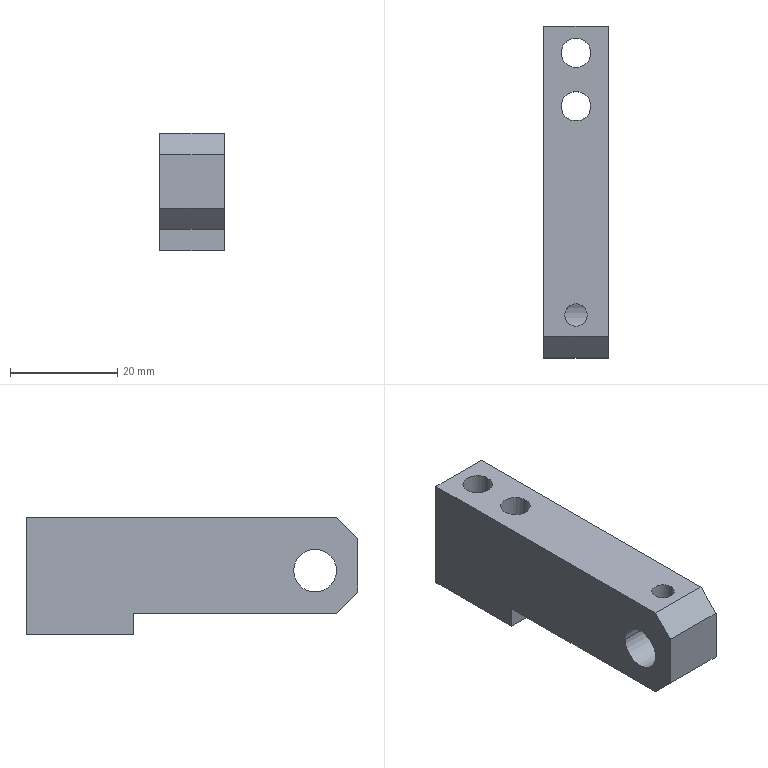Component | SolidWorks | STB-08-009-2 | 1 solid | 18 faces | box 12 x 62 x 22 mm | volume 12426 mm3 | plane 10 | cylinder 8 | commonest cylinder face diameters 5.5 x4 4.2 x2 8 x2
build123d program:
from build123d import *

# Parameters (mm, degrees)
SKETCH1_W                  = 12
SKETCH1_H                  = 62
BOSS_EXTRUDE1_DEPTH        = 11
CUT_EXTRUDE1_REACH         = 37.014
SKETCH2_W                  = 4
SKETCH2_H                  = 42
F_5_5_5_5_DIAMETER_HOLE1_D = 5.5
CUT_EXTRUDE2_REACH         = 37.014
SKETCH5_R                  = 4
M5_TAPPED_HOLE1_REACH      = 40.484
M5_TAPPED_HOLE1_BORE_R     = 2.1
CHAMFER1_SIZE              = 4


with BuildPart() as part:
    # Sketch1 → Boss-Extrude1 (new, symmetric)
    with BuildSketch(Plane.XY):
        Rectangle(SKETCH1_W, SKETCH1_H)
    extrude(amount=BOSS_EXTRUDE1_DEPTH, both=True)

    # Sketch2 → Cut-Extrude1 (cut, up to next)
    with BuildSketch(Plane(origin=(6, 0, 0), x_dir=(0, 0, -1), z_dir=(1, 0, 0)), mode=Mode.PRIVATE) as cut_extrude1_sk1:
        with Locations((9, -10)):
            Rectangle(SKETCH2_W, SKETCH2_H)
    cut_extrude1_tool1 = extrude(cut_extrude1_sk1.sketch, amount=-CUT_EXTRUDE1_REACH, mode=Mode.PRIVATE) & part.part
    add(cut_extrude1_tool1.solids().sort_by_distance((6, -10, -9))[0], mode=Mode.SUBTRACT)

    # 5.5 _5.5_ Diameter Hole1 (through all)
    with Locations(Plane.XY.offset(11)):
        with Locations((0, 26), (0, 16)):
            Hole(F_5_5_5_5_DIAMETER_HOLE1_D / 2)

    # Sketch5 → Cut-Extrude2 (cut, up to next)
    with BuildSketch(Plane(origin=(6, 0, 0), x_dir=(0, 0, -1), z_dir=(1, 0, 0)), mode=Mode.PRIVATE) as cut_extrude2_sk1:
        with Locations(Location((-1, -23, 0), (0, 0, 90))):
            Circle(SKETCH5_R)
    cut_extrude2_tool1 = extrude(cut_extrude2_sk1.sketch, amount=-CUT_EXTRUDE2_REACH, mode=Mode.PRIVATE) & part.part
    add(cut_extrude2_tool1.solids().sort_by_distance((6, -23, 1))[0], mode=Mode.SUBTRACT)

    # M5 Tapped Hole1 bore → M5 Tapped Hole1 (cut, up to next)
    with BuildSketch(Plane.XY.offset(11), mode=Mode.PRIVATE) as m5_tapped_hole1_sk1:
        with Locations((0, -23)):
            Circle(M5_TAPPED_HOLE1_BORE_R)
    m5_tapped_hole1_tool1 = extrude(m5_tapped_hole1_sk1.sketch, amount=-M5_TAPPED_HOLE1_REACH, mode=Mode.PRIVATE) & part.part
    add(m5_tapped_hole1_tool1.solids().sort_by_distance((0, -23, 11))[0], mode=Mode.SUBTRACT)

    # Chamfer1
    chamfer1_edges = [part.edges().sort_by_distance(p)[0] for p in [
        (0, -31, -7),
        (0, -31, 11),
    ]]
    chamfer(chamfer1_edges, length=CHAMFER1_SIZE)


solid = part.part

# Placed as in the assembly
solid = solid.moved(Location((10.096, 88.999, -20), (0, 0, 0)))
STEP:
#1=COLOUR_RGB('',0.7922,0.8196,0.9333);
#2=FILL_AREA_STYLE_COLOUR('',#1);
#3=FILL_AREA_STYLE('',(#2));
#4=SURFACE_STYLE_FILL_AREA(#3);
#5=SURFACE_SIDE_STYLE('',(#4));
#6=SURFACE_STYLE_USAGE(.BOTH.,#5);
#7=PRESENTATION_STYLE_ASSIGNMENT((#6));
#8=CARTESIAN_POINT('',(0.3148,2.598,-0.5906));
#9=VERTEX_POINT('',#8);
#10=CARTESIAN_POINT('',(0.4802,2.598,-0.5906));
#11=VERTEX_POINT('',#10);
#12=CARTESIAN_POINT('',(0.3148,2.598,-0.5906));
#13=CARTESIAN_POINT('',(0.3148,2.593,-0.5906));
#14=CARTESIAN_POINT('',(0.3154,2.587,-0.5908));
#15=CARTESIAN_POINT('',(0.3176,2.577,-0.592));
#16=CARTESIAN_POINT('',(0.3192,2.571,-0.5928));
#17=CARTESIAN_POINT('',(0.3234,2.561,-0.5949));
#18=CARTESIAN_POINT('',(0.326,2.557,-0.5961));
#19=CARTESIAN_POINT('',(0.3319,2.548,-0.5988));
#20=CARTESIAN_POINT('',(0.3354,2.544,-0.6003));
#21=CARTESIAN_POINT('',(0.3429,2.536,-0.6033));
#22=CARTESIAN_POINT('',(0.347,2.533,-0.6048));
#23=CARTESIAN_POINT('',(0.3558,2.527,-0.6077));
#24=CARTESIAN_POINT('',(0.3606,2.524,-0.6091));
#25=CARTESIAN_POINT('',(0.3754,2.518,-0.6125));
#26=CARTESIAN_POINT('',(0.3864,2.516,-0.614));
#27=CARTESIAN_POINT('',(0.4029,2.516,-0.614));
#28=CARTESIAN_POINT('',(0.4084,2.516,-0.6137));
#29=CARTESIAN_POINT('',(0.4192,2.518,-0.6124));
#30=CARTESIAN_POINT('',(0.4244,2.52,-0.6114));
#31=CARTESIAN_POINT('',(0.4344,2.524,-0.6091));
#32=CARTESIAN_POINT('',(0.4391,2.527,-0.6077));
#33=CARTESIAN_POINT('',(0.448,2.533,-0.6049));
#34=CARTESIAN_POINT('',(0.4521,2.536,-0.6033));
#35=CARTESIAN_POINT('',(0.4596,2.544,-0.6003));
#36=CARTESIAN_POINT('',(0.463,2.548,-0.5989));
#37=CARTESIAN_POINT('',(0.469,2.557,-0.5961));
#38=CARTESIAN_POINT('',(0.4716,2.561,-0.5949));
#39=CARTESIAN_POINT('',(0.4758,2.571,-0.5928));
#40=CARTESIAN_POINT('',(0.4774,2.576,-0.592));
#41=CARTESIAN_POINT('',(0.4796,2.587,-0.5909));
#42=CARTESIAN_POINT('',(0.4802,2.593,-0.5906));
#43=CARTESIAN_POINT('',(0.4802,2.598,-0.5906));
#44=B_SPLINE_CURVE_WITH_KNOTS('',3,(#12,#13,#14,#15,#16,#17,#18,#19,#20,#21,#22,#23,#24,#25,#26,#27,#28,#29,#30,#31,#32,#33,#34,#35,#36,#37,#38,#39,#40,#41,#42,#43),.UNSPECIFIED.,.F.,.F.,(4,2,2,2,2,2,2,2,2,2,2,2,2,2,2,4),(0.006693,0.007111,0.007528,0.007946,0.008363,0.008781,0.009198,0.01003,0.01045,0.01087,0.01129,0.0117,0.01212,0.01254,0.01296,0.01337),.UNSPECIFIED.);
#45=EDGE_CURVE('',#9,#11,#44,.T.);
#46=ORIENTED_EDGE('',*,*,#45,.F.);
#47=CARTESIAN_POINT('',(0.3148,2.598,-0.3543));
#48=VERTEX_POINT('',#47);
#49=CARTESIAN_POINT('',(0.3148,2.598,-0.3543));
#50=DIRECTION('',(0.,0.,1.));
#51=VECTOR('',#50,39.37);
#52=LINE('',#49,#51);
#53=EDGE_CURVE('',#9,#48,#52,.T.);
#54=ORIENTED_EDGE('',*,*,#53,.T.);
#55=CARTESIAN_POINT('',(0.4802,2.598,-0.3543));
#56=VERTEX_POINT('',#55);
#57=CARTESIAN_POINT('',(0.3975,2.598,-0.3543));
#58=DIRECTION('',(0.,0.,1.));
#59=DIRECTION('',(1.,0.,0.));
#60=AXIS2_PLACEMENT_3D('',#57,#58,#59);
#61=CIRCLE('',#60,0.08268);
#62=EDGE_CURVE('',#48,#56,#61,.T.);
#63=ORIENTED_EDGE('',*,*,#62,.T.);
#64=CARTESIAN_POINT('',(0.4802,2.598,-0.3543));
#65=DIRECTION('',(0.,0.,1.));
#66=VECTOR('',#65,39.37);
#67=LINE('',#64,#66);
#68=EDGE_CURVE('',#11,#56,#67,.T.);
#69=ORIENTED_EDGE('',*,*,#68,.F.);
#70=EDGE_LOOP('',(#46,#54,#63,#69));
#71=FACE_OUTER_BOUND('',#70,.T.);
#72=CARTESIAN_POINT('',(0.3975,2.598,-0.3543));
#73=DIRECTION('',(0.,0.,1.));
#74=DIRECTION('',(1.,0.,0.));
#75=AXIS2_PLACEMENT_3D('',#72,#73,#74);
#76=CYLINDRICAL_SURFACE('',#75,0.08268);
#77=ADVANCED_FACE('',(#71),#76,.F.);
#78=CARTESIAN_POINT('',(0.1613,2.756,-0.748));
#79=VERTEX_POINT('',#78);
#80=CARTESIAN_POINT('',(0.1613,2.441,-0.748));
#81=VERTEX_POINT('',#80);
#82=CARTESIAN_POINT('',(0.1613,2.598,-0.748));
#83=DIRECTION('',(-1.,0.,0.));
#84=DIRECTION('',(0.,0.,-1.));
#85=AXIS2_PLACEMENT_3D('',#82,#83,#84);
#86=CIRCLE('',#85,0.1575);
#87=EDGE_CURVE('',#79,#81,#86,.T.);
#88=ORIENTED_EDGE('',*,*,#87,.T.);
#89=CARTESIAN_POINT('',(0.6337,2.441,-0.748));
#90=VERTEX_POINT('',#89);
#91=CARTESIAN_POINT('',(0.1612,2.441,-0.748));
#92=DIRECTION('',(1.,0.,0.));
#93=VECTOR('',#92,39.37);
#94=LINE('',#91,#93);
#95=EDGE_CURVE('',#81,#90,#94,.T.);
#96=ORIENTED_EDGE('',*,*,#95,.T.);
#97=CARTESIAN_POINT('',(0.6337,2.756,-0.748));
#98=VERTEX_POINT('',#97);
#99=CARTESIAN_POINT('',(0.6337,2.598,-0.748));
#100=DIRECTION('',(1.,0.,0.));
#101=DIRECTION('',(0.,1.,0.));
#102=AXIS2_PLACEMENT_3D('',#99,#100,#101);
#103=CIRCLE('',#102,0.1575);
#104=EDGE_CURVE('',#90,#98,#103,.T.);
#105=ORIENTED_EDGE('',*,*,#104,.T.);
#106=CARTESIAN_POINT('',(0.1612,2.756,-0.748));
#107=DIRECTION('',(1.,0.,0.));
#108=VECTOR('',#107,39.37);
#109=LINE('',#106,#108);
#110=EDGE_CURVE('',#79,#98,#109,.T.);
#111=ORIENTED_EDGE('',*,*,#110,.F.);
#112=EDGE_LOOP('',(#88,#96,#105,#111));
#113=FACE_OUTER_BOUND('',#112,.T.);
#114=CARTESIAN_POINT('',(0.1612,2.598,-0.748));
#115=DIRECTION('',(1.,0.,0.));
#116=DIRECTION('',(0.,1.,0.));
#117=AXIS2_PLACEMENT_3D('',#114,#115,#116);
#118=CYLINDRICAL_SURFACE('',#117,0.1575);
#119=ADVANCED_FACE('',(#113),#118,.F.);
#120=CARTESIAN_POINT('',(0.2892,4.528,-1.22));
#121=VERTEX_POINT('',#120);
#122=CARTESIAN_POINT('',(0.5058,4.528,-1.22));
#123=VERTEX_POINT('',#122);
#124=CARTESIAN_POINT('',(0.3975,4.528,-1.22));
#125=DIRECTION('',(0.,0.,1.));
#126=DIRECTION('',(1.,0.,0.));
#127=AXIS2_PLACEMENT_3D('',#124,#125,#126);
#128=CIRCLE('',#127,0.1083);
#129=EDGE_CURVE('',#121,#123,#128,.T.);
#130=ORIENTED_EDGE('',*,*,#129,.F.);
#131=CARTESIAN_POINT('',(0.2892,4.528,-0.3543));
#132=VERTEX_POINT('',#131);
#133=CARTESIAN_POINT('',(0.2892,4.528,-0.3543));
#134=DIRECTION('',(0.,0.,1.));
#135=VECTOR('',#134,39.37);
#136=LINE('',#133,#135);
#137=EDGE_CURVE('',#121,#132,#136,.T.);
#138=ORIENTED_EDGE('',*,*,#137,.T.);
#139=CARTESIAN_POINT('',(0.5058,4.528,-0.3543));
#140=VERTEX_POINT('',#139);
#141=CARTESIAN_POINT('',(0.3975,4.528,-0.3543));
#142=DIRECTION('',(0.,0.,1.));
#143=DIRECTION('',(1.,0.,0.));
#144=AXIS2_PLACEMENT_3D('',#141,#142,#143);
#145=CIRCLE('',#144,0.1083);
#146=EDGE_CURVE('',#132,#140,#145,.T.);
#147=ORIENTED_EDGE('',*,*,#146,.T.);
#148=CARTESIAN_POINT('',(0.5058,4.528,-0.3543));
#149=DIRECTION('',(0.,0.,1.));
#150=VECTOR('',#149,39.37);
#151=LINE('',#148,#150);
#152=EDGE_CURVE('',#123,#140,#151,.T.);
#153=ORIENTED_EDGE('',*,*,#152,.F.);
#154=EDGE_LOOP('',(#130,#138,#147,#153));
#155=FACE_OUTER_BOUND('',#154,.T.);
#156=CARTESIAN_POINT('',(0.3975,4.528,-0.3543));
#157=DIRECTION('',(0.,0.,1.));
#158=DIRECTION('',(1.,0.,0.));
#159=AXIS2_PLACEMENT_3D('',#156,#157,#158);
#160=CYLINDRICAL_SURFACE('',#159,0.1083);
#161=ADVANCED_FACE('',(#155),#160,.F.);
#162=CARTESIAN_POINT('',(0.2892,4.134,-1.22));
#163=VERTEX_POINT('',#162);
#164=CARTESIAN_POINT('',(0.5058,4.134,-1.22));
#165=VERTEX_POINT('',#164);
#166=CARTESIAN_POINT('',(0.3975,4.134,-1.22));
#167=DIRECTION('',(0.,0.,1.));
#168=DIRECTION('',(1.,0.,0.));
#169=AXIS2_PLACEMENT_3D('',#166,#167,#168);
#170=CIRCLE('',#169,0.1083);
#171=EDGE_CURVE('',#163,#165,#170,.T.);
#172=ORIENTED_EDGE('',*,*,#171,.F.);
#173=CARTESIAN_POINT('',(0.2892,4.134,-0.3543));
#174=VERTEX_POINT('',#173);
#175=CARTESIAN_POINT('',(0.2892,4.134,-0.3543));
#176=DIRECTION('',(0.,0.,1.));
#177=VECTOR('',#176,39.37);
#178=LINE('',#175,#177);
#179=EDGE_CURVE('',#163,#174,#178,.T.);
#180=ORIENTED_EDGE('',*,*,#179,.T.);
#181=CARTESIAN_POINT('',(0.5058,4.134,-0.3543));
#182=VERTEX_POINT('',#181);
#183=CARTESIAN_POINT('',(0.3975,4.134,-0.3543));
#184=DIRECTION('',(0.,0.,1.));
#185=DIRECTION('',(1.,0.,0.));
#186=AXIS2_PLACEMENT_3D('',#183,#184,#185);
#187=CIRCLE('',#186,0.1083);
#188=EDGE_CURVE('',#174,#182,#187,.T.);
#189=ORIENTED_EDGE('',*,*,#188,.T.);
#190=CARTESIAN_POINT('',(0.5058,4.134,-0.3543));
#191=DIRECTION('',(0.,0.,1.));
#192=VECTOR('',#191,39.37);
#193=LINE('',#190,#192);
#194=EDGE_CURVE('',#165,#182,#193,.T.);
#195=ORIENTED_EDGE('',*,*,#194,.F.);
#196=EDGE_LOOP('',(#172,#180,#189,#195));
#197=FACE_OUTER_BOUND('',#196,.T.);
#198=CARTESIAN_POINT('',(0.3975,4.134,-0.3543));
#199=DIRECTION('',(0.,0.,1.));
#200=DIRECTION('',(1.,0.,0.));
#201=AXIS2_PLACEMENT_3D('',#198,#199,#200);
#202=CYLINDRICAL_SURFACE('',#201,0.1083);
#203=ADVANCED_FACE('',(#197),#202,.F.);
#204=ORIENTED_EDGE('',*,*,#87,.F.);
#205=CARTESIAN_POINT('',(0.1613,2.598,-0.748));
#206=DIRECTION('',(-1.,0.,0.));
#207=DIRECTION('',(0.,0.,-1.));
#208=AXIS2_PLACEMENT_3D('',#205,#206,#207);
#209=CIRCLE('',#208,0.1575);
#210=EDGE_CURVE('',#81,#79,#209,.T.);
#211=ORIENTED_EDGE('',*,*,#210,.F.);
#212=EDGE_LOOP('',(#204,#211));
#213=FACE_BOUND('',#212,.T.);
#214=CARTESIAN_POINT('',(0.1613,2.441,-1.063));
#215=VERTEX_POINT('',#214);
#216=CARTESIAN_POINT('',(0.1613,3.937,-1.063));
#217=VERTEX_POINT('',#216);
#218=CARTESIAN_POINT('',(0.1613,2.283,-1.063));
#219=DIRECTION('',(0.,1.,-0.));
#220=VECTOR('',#219,39.37);
#221=LINE('',#218,#220);
#222=EDGE_CURVE('',#215,#217,#221,.T.);
#223=ORIENTED_EDGE('',*,*,#222,.F.);
#224=CARTESIAN_POINT('',(0.1613,2.283,-0.9055));
#225=VERTEX_POINT('',#224);
#226=CARTESIAN_POINT('',(0.1613,2.283,-0.9055));
#227=DIRECTION('',(0.,-0.7071,0.7071));
#228=VECTOR('',#227,39.37);
#229=LINE('',#226,#228);
#230=EDGE_CURVE('',#215,#225,#229,.T.);
#231=ORIENTED_EDGE('',*,*,#230,.T.);
#232=CARTESIAN_POINT('',(0.1613,2.283,-0.5118));
#233=VERTEX_POINT('',#232);
#234=CARTESIAN_POINT('',(0.1613,2.283,-0.3543));
#235=DIRECTION('',(0.,0.,-1.));
#236=VECTOR('',#235,39.37);
#237=LINE('',#234,#236);
#238=EDGE_CURVE('',#233,#225,#237,.T.);
#239=ORIENTED_EDGE('',*,*,#238,.F.);
#240=CARTESIAN_POINT('',(0.1613,2.441,-0.3543));
#241=VERTEX_POINT('',#240);
#242=CARTESIAN_POINT('',(0.1613,2.441,-0.3543));
#243=DIRECTION('',(0.,0.7071,0.7071));
#244=VECTOR('',#243,39.37);
#245=LINE('',#242,#244);
#246=EDGE_CURVE('',#233,#241,#245,.T.);
#247=ORIENTED_EDGE('',*,*,#246,.T.);
#248=CARTESIAN_POINT('',(0.1613,4.724,-0.3543));
#249=VERTEX_POINT('',#248);
#250=CARTESIAN_POINT('',(0.1613,4.724,-0.3543));
#251=DIRECTION('',(0.,-1.,0.));
#252=VECTOR('',#251,39.37);
#253=LINE('',#250,#252);
#254=EDGE_CURVE('',#249,#241,#253,.T.);
#255=ORIENTED_EDGE('',*,*,#254,.F.);
#256=CARTESIAN_POINT('',(0.1613,4.724,-1.22));
#257=VERTEX_POINT('',#256);
#258=CARTESIAN_POINT('',(0.1613,4.724,-0.3543));
#259=DIRECTION('',(0.,0.,-1.));
#260=VECTOR('',#259,39.37);
#261=LINE('',#258,#260);
#262=EDGE_CURVE('',#249,#257,#261,.T.);
#263=ORIENTED_EDGE('',*,*,#262,.T.);
#264=CARTESIAN_POINT('',(0.1613,3.937,-1.22));
#265=VERTEX_POINT('',#264);
#266=CARTESIAN_POINT('',(0.1613,4.724,-1.22));
#267=DIRECTION('',(0.,-1.,0.));
#268=VECTOR('',#267,39.37);
#269=LINE('',#266,#268);
#270=EDGE_CURVE('',#257,#265,#269,.T.);
#271=ORIENTED_EDGE('',*,*,#270,.T.);
#272=CARTESIAN_POINT('',(0.1613,3.937,-1.22));
#273=DIRECTION('',(0.,0.,-1.));
#274=VECTOR('',#273,39.37);
#275=LINE('',#272,#274);
#276=EDGE_CURVE('',#217,#265,#275,.T.);
#277=ORIENTED_EDGE('',*,*,#276,.F.);
#278=EDGE_LOOP('',(#223,#231,#239,#247,#255,#263,#271,#277));
#279=FACE_OUTER_BOUND('',#278,.T.);
#280=CARTESIAN_POINT('',(0.1613,4.724,-0.3543));
#281=DIRECTION('',(1.,0.,0.));
#282=DIRECTION('',(0.,0.,-1.));
#283=AXIS2_PLACEMENT_3D('',#280,#281,#282);
#284=PLANE('',#283);
#285=ADVANCED_FACE('',(#213,#279),#284,.F.);
#286=ORIENTED_EDGE('',*,*,#238,.T.);
#287=CARTESIAN_POINT('',(0.6337,2.283,-0.9055));
#288=VERTEX_POINT('',#287);
#289=CARTESIAN_POINT('',(0.1613,2.283,-0.9055));
#290=DIRECTION('',(1.,0.,0.));
#291=VECTOR('',#290,39.37);
#292=LINE('',#289,#291);
#293=EDGE_CURVE('',#225,#288,#292,.T.);
#294=ORIENTED_EDGE('',*,*,#293,.T.);
#295=CARTESIAN_POINT('',(0.6337,2.283,-0.5118));
#296=VERTEX_POINT('',#295);
#297=CARTESIAN_POINT('',(0.6337,2.283,-0.3543));
#298=DIRECTION('',(0.,0.,-1.));
#299=VECTOR('',#298,39.37);
#300=LINE('',#297,#299);
#301=EDGE_CURVE('',#296,#288,#300,.T.);
#302=ORIENTED_EDGE('',*,*,#301,.F.);
#303=CARTESIAN_POINT('',(0.1613,2.283,-0.5118));
#304=DIRECTION('',(-1.,0.,0.));
#305=VECTOR('',#304,39.37);
#306=LINE('',#303,#305);
#307=EDGE_CURVE('',#296,#233,#306,.T.);
#308=ORIENTED_EDGE('',*,*,#307,.T.);
#309=EDGE_LOOP('',(#286,#294,#302,#308));
#310=FACE_OUTER_BOUND('',#309,.T.);
#311=CARTESIAN_POINT('',(0.1613,2.283,-0.3543));
#312=DIRECTION('',(0.,1.,0.));
#313=DIRECTION('',(0.,0.,1.));
#314=AXIS2_PLACEMENT_3D('',#311,#312,#313);
#315=PLANE('',#314);
#316=ADVANCED_FACE('',(#310),#315,.F.);
#317=CARTESIAN_POINT('',(0.6337,2.598,-0.748));
#318=DIRECTION('',(1.,0.,0.));
#319=DIRECTION('',(0.,1.,0.));
#320=AXIS2_PLACEMENT_3D('',#317,#318,#319);
#321=CIRCLE('',#320,0.1575);
#322=EDGE_CURVE('',#98,#90,#321,.T.);
#323=ORIENTED_EDGE('',*,*,#322,.F.);
#324=ORIENTED_EDGE('',*,*,#104,.F.);
#325=EDGE_LOOP('',(#323,#324));
#326=FACE_BOUND('',#325,.T.);
#327=ORIENTED_EDGE('',*,*,#301,.T.);
#328=CARTESIAN_POINT('',(0.6337,2.441,-1.063));
#329=VERTEX_POINT('',#328);
#330=CARTESIAN_POINT('',(0.6337,2.283,-0.9055));
#331=DIRECTION('',(0.,0.7071,-0.7071));
#332=VECTOR('',#331,39.37);
#333=LINE('',#330,#332);
#334=EDGE_CURVE('',#288,#329,#333,.T.);
#335=ORIENTED_EDGE('',*,*,#334,.T.);
#336=CARTESIAN_POINT('',(0.6337,3.937,-1.063));
#337=VERTEX_POINT('',#336);
#338=CARTESIAN_POINT('',(0.6337,2.283,-1.063));
#339=DIRECTION('',(0.,-1.,0.));
#340=VECTOR('',#339,39.37);
#341=LINE('',#338,#340);
#342=EDGE_CURVE('',#337,#329,#341,.T.);
#343=ORIENTED_EDGE('',*,*,#342,.F.);
#344=CARTESIAN_POINT('',(0.6337,3.937,-1.22));
#345=VERTEX_POINT('',#344);
#346=CARTESIAN_POINT('',(0.6337,3.937,-1.22));
#347=DIRECTION('',(0.,0.,1.));
#348=VECTOR('',#347,39.37);
#349=LINE('',#346,#348);
#350=EDGE_CURVE('',#345,#337,#349,.T.);
#351=ORIENTED_EDGE('',*,*,#350,.F.);
#352=CARTESIAN_POINT('',(0.6337,4.724,-1.22));
#353=VERTEX_POINT('',#352);
#354=CARTESIAN_POINT('',(0.6337,4.724,-1.22));
#355=DIRECTION('',(0.,1.,0.));
#356=VECTOR('',#355,39.37);
#357=LINE('',#354,#356);
#358=EDGE_CURVE('',#345,#353,#357,.T.);
#359=ORIENTED_EDGE('',*,*,#358,.T.);
#360=CARTESIAN_POINT('',(0.6337,4.724,-0.3543));
#361=VERTEX_POINT('',#360);
#362=CARTESIAN_POINT('',(0.6337,4.724,-0.3543));
#363=DIRECTION('',(0.,0.,-1.));
#364=VECTOR('',#363,39.37);
#365=LINE('',#362,#364);
#366=EDGE_CURVE('',#361,#353,#365,.T.);
#367=ORIENTED_EDGE('',*,*,#366,.F.);
#368=CARTESIAN_POINT('',(0.6337,2.441,-0.3543));
#369=VERTEX_POINT('',#368);
#370=CARTESIAN_POINT('',(0.6337,4.724,-0.3543));
#371=DIRECTION('',(0.,1.,0.));
#372=VECTOR('',#371,39.37);
#373=LINE('',#370,#372);
#374=EDGE_CURVE('',#369,#361,#373,.T.);
#375=ORIENTED_EDGE('',*,*,#374,.F.);
#376=CARTESIAN_POINT('',(0.6337,2.441,-0.3543));
#377=DIRECTION('',(0.,-0.7071,-0.7071));
#378=VECTOR('',#377,39.37);
#379=LINE('',#376,#378);
#380=EDGE_CURVE('',#369,#296,#379,.T.);
#381=ORIENTED_EDGE('',*,*,#380,.T.);
#382=EDGE_LOOP('',(#327,#335,#343,#351,#359,#367,#375,#381));
#383=FACE_OUTER_BOUND('',#382,.T.);
#384=CARTESIAN_POINT('',(0.6337,4.724,-0.3543));
#385=DIRECTION('',(-1.,0.,0.));
#386=DIRECTION('',(0.,0.,1.));
#387=AXIS2_PLACEMENT_3D('',#384,#385,#386);
#388=PLANE('',#387);
#389=ADVANCED_FACE('',(#326,#383),#388,.F.);
#390=CARTESIAN_POINT('',(0.1613,4.724,-1.22));
#391=DIRECTION('',(-1.,0.,0.));
#392=VECTOR('',#391,39.37);
#393=LINE('',#390,#392);
#394=EDGE_CURVE('',#353,#257,#393,.T.);
#395=ORIENTED_EDGE('',*,*,#394,.T.);
#396=ORIENTED_EDGE('',*,*,#262,.F.);
#397=CARTESIAN_POINT('',(0.1613,4.724,-0.3543));
#398=DIRECTION('',(-1.,0.,0.));
#399=VECTOR('',#398,39.37);
#400=LINE('',#397,#399);
#401=EDGE_CURVE('',#361,#249,#400,.T.);
#402=ORIENTED_EDGE('',*,*,#401,.F.);
#403=ORIENTED_EDGE('',*,*,#366,.T.);
#404=EDGE_LOOP('',(#395,#396,#402,#403));
#405=FACE_OUTER_BOUND('',#404,.T.);
#406=CARTESIAN_POINT('',(0.1613,4.724,-0.3543));
#407=DIRECTION('',(0.,-1.,0.));
#408=DIRECTION('',(0.,0.,-1.));
#409=AXIS2_PLACEMENT_3D('',#406,#407,#408);
#410=PLANE('',#409);
#411=ADVANCED_FACE('',(#405),#410,.F.);
#412=CARTESIAN_POINT('',(0.3975,2.598,-0.3543));
#413=DIRECTION('',(0.,0.,1.));
#414=DIRECTION('',(1.,0.,0.));
#415=AXIS2_PLACEMENT_3D('',#412,#413,#414);
#416=CIRCLE('',#415,0.08268);
#417=EDGE_CURVE('',#56,#48,#416,.T.);
#418=ORIENTED_EDGE('',*,*,#417,.F.);
#419=ORIENTED_EDGE('',*,*,#62,.F.);
#420=EDGE_LOOP('',(#418,#419));
#421=FACE_BOUND('',#420,.T.);
#422=CARTESIAN_POINT('',(0.3975,4.528,-0.3543));
#423=DIRECTION('',(0.,0.,1.));
#424=DIRECTION('',(1.,0.,0.));
#425=AXIS2_PLACEMENT_3D('',#422,#423,#424);
#426=CIRCLE('',#425,0.1083);
#427=EDGE_CURVE('',#140,#132,#426,.T.);
#428=ORIENTED_EDGE('',*,*,#427,.F.);
#429=ORIENTED_EDGE('',*,*,#146,.F.);
#430=EDGE_LOOP('',(#428,#429));
#431=FACE_BOUND('',#430,.T.);
#432=CARTESIAN_POINT('',(0.3975,4.134,-0.3543));
#433=DIRECTION('',(0.,0.,1.));
#434=DIRECTION('',(1.,0.,0.));
#435=AXIS2_PLACEMENT_3D('',#432,#433,#434);
#436=CIRCLE('',#435,0.1083);
#437=EDGE_CURVE('',#182,#174,#436,.T.);
#438=ORIENTED_EDGE('',*,*,#437,.F.);
#439=ORIENTED_EDGE('',*,*,#188,.F.);
#440=EDGE_LOOP('',(#438,#439));
#441=FACE_BOUND('',#440,.T.);
#442=ORIENTED_EDGE('',*,*,#254,.T.);
#443=CARTESIAN_POINT('',(0.6337,2.441,-0.3543));
#444=DIRECTION('',(1.,0.,0.));
#445=VECTOR('',#444,39.37);
#446=LINE('',#443,#445);
#447=EDGE_CURVE('',#241,#369,#446,.T.);
#448=ORIENTED_EDGE('',*,*,#447,.T.);
#449=ORIENTED_EDGE('',*,*,#374,.T.);
#450=ORIENTED_EDGE('',*,*,#401,.T.);
#451=EDGE_LOOP('',(#442,#448,#449,#450));
#452=FACE_OUTER_BOUND('',#451,.T.);
#453=CARTESIAN_POINT('',(0.1613,2.283,-0.3543));
#454=DIRECTION('',(0.,0.,1.));
#455=DIRECTION('',(1.,0.,0.));
#456=AXIS2_PLACEMENT_3D('',#453,#454,#455);
#457=PLANE('',#456);
#458=ADVANCED_FACE('',(#421,#431,#441,#452),#457,.T.);
#459=CARTESIAN_POINT('',(0.3975,4.528,-1.22));
#460=DIRECTION('',(0.,0.,1.));
#461=DIRECTION('',(1.,0.,0.));
#462=AXIS2_PLACEMENT_3D('',#459,#460,#461);
#463=CIRCLE('',#462,0.1083);
#464=EDGE_CURVE('',#123,#121,#463,.T.);
#465=ORIENTED_EDGE('',*,*,#464,.T.);
#466=ORIENTED_EDGE('',*,*,#129,.T.);
#467=EDGE_LOOP('',(#465,#466));
#468=FACE_BOUND('',#467,.T.);
#469=CARTESIAN_POINT('',(0.3975,4.134,-1.22));
#470=DIRECTION('',(0.,0.,1.));
#471=DIRECTION('',(1.,0.,0.));
#472=AXIS2_PLACEMENT_3D('',#469,#470,#471);
#473=CIRCLE('',#472,0.1083);
#474=EDGE_CURVE('',#165,#163,#473,.T.);
#475=ORIENTED_EDGE('',*,*,#474,.T.);
#476=ORIENTED_EDGE('',*,*,#171,.T.);
#477=EDGE_LOOP('',(#475,#476));
#478=FACE_BOUND('',#477,.T.);
#479=ORIENTED_EDGE('',*,*,#358,.F.);
#480=CARTESIAN_POINT('',(0.1612,3.937,-1.22));
#481=DIRECTION('',(1.,0.,0.));
#482=VECTOR('',#481,39.37);
#483=LINE('',#480,#482);
#484=EDGE_CURVE('',#265,#345,#483,.T.);
#485=ORIENTED_EDGE('',*,*,#484,.F.);
#486=ORIENTED_EDGE('',*,*,#270,.F.);
#487=ORIENTED_EDGE('',*,*,#394,.F.);
#488=EDGE_LOOP('',(#479,#485,#486,#487));
#489=FACE_OUTER_BOUND('',#488,.T.);
#490=CARTESIAN_POINT('',(0.1613,2.283,-1.22));
#491=DIRECTION('',(0.,0.,1.));
#492=DIRECTION('',(1.,0.,0.));
#493=AXIS2_PLACEMENT_3D('',#490,#491,#492);
#494=PLANE('',#493);
#495=ADVANCED_FACE('',(#468,#478,#489),#494,.F.);
#496=ORIENTED_EDGE('',*,*,#342,.T.);
#497=CARTESIAN_POINT('',(0.1612,2.441,-1.063));
#498=DIRECTION('',(-1.,0.,-0.));
#499=VECTOR('',#498,39.37);
#500=LINE('',#497,#499);
#501=EDGE_CURVE('',#329,#215,#500,.T.);
#502=ORIENTED_EDGE('',*,*,#501,.T.);
#503=ORIENTED_EDGE('',*,*,#222,.T.);
#504=CARTESIAN_POINT('',(0.1612,3.937,-1.063));
#505=DIRECTION('',(1.,0.,0.));
#506=VECTOR('',#505,39.37);
#507=LINE('',#504,#506);
#508=EDGE_CURVE('',#217,#337,#507,.T.);
#509=ORIENTED_EDGE('',*,*,#508,.T.);
#510=EDGE_LOOP('',(#496,#502,#503,#509));
#511=FACE_OUTER_BOUND('',#510,.T.);
#512=CARTESIAN_POINT('',(0.1612,2.283,-1.063));
#513=DIRECTION('',(-0.,0.,1.));
#514=DIRECTION('',(0.,-1.,0.));
#515=AXIS2_PLACEMENT_3D('',#512,#513,#514);
#516=PLANE('',#515);
#517=ADVANCED_FACE('',(#511),#516,.F.);
#518=ORIENTED_EDGE('',*,*,#276,.T.);
#519=ORIENTED_EDGE('',*,*,#484,.T.);
#520=ORIENTED_EDGE('',*,*,#350,.T.);
#521=ORIENTED_EDGE('',*,*,#508,.F.);
#522=EDGE_LOOP('',(#518,#519,#520,#521));
#523=FACE_OUTER_BOUND('',#522,.T.);
#524=CARTESIAN_POINT('',(0.1612,3.937,-1.22));
#525=DIRECTION('',(-0.,1.,0.));
#526=DIRECTION('',(-1.,-0.,0.));
#527=AXIS2_PLACEMENT_3D('',#524,#525,#526);
#528=PLANE('',#527);
#529=ADVANCED_FACE('',(#523),#528,.F.);
#530=ORIENTED_EDGE('',*,*,#179,.F.);
#531=ORIENTED_EDGE('',*,*,#474,.F.);
#532=ORIENTED_EDGE('',*,*,#194,.T.);
#533=ORIENTED_EDGE('',*,*,#437,.T.);
#534=EDGE_LOOP('',(#530,#531,#532,#533));
#535=FACE_OUTER_BOUND('',#534,.T.);
#536=CARTESIAN_POINT('',(0.3975,4.134,-0.3543));
#537=DIRECTION('',(0.,0.,1.));
#538=DIRECTION('',(1.,0.,0.));
#539=AXIS2_PLACEMENT_3D('',#536,#537,#538);
#540=CYLINDRICAL_SURFACE('',#539,0.1083);
#541=ADVANCED_FACE('',(#535),#540,.F.);
#542=ORIENTED_EDGE('',*,*,#137,.F.);
#543=ORIENTED_EDGE('',*,*,#464,.F.);
#544=ORIENTED_EDGE('',*,*,#152,.T.);
#545=ORIENTED_EDGE('',*,*,#427,.T.);
#546=EDGE_LOOP('',(#542,#543,#544,#545));
#547=FACE_OUTER_BOUND('',#546,.T.);
#548=CARTESIAN_POINT('',(0.3975,4.528,-0.3543));
#549=DIRECTION('',(0.,0.,1.));
#550=DIRECTION('',(1.,0.,0.));
#551=AXIS2_PLACEMENT_3D('',#548,#549,#550);
#552=CYLINDRICAL_SURFACE('',#551,0.1083);
#553=ADVANCED_FACE('',(#547),#552,.F.);
#554=ORIENTED_EDGE('',*,*,#95,.F.);
#555=ORIENTED_EDGE('',*,*,#210,.T.);
#556=ORIENTED_EDGE('',*,*,#110,.T.);
#557=ORIENTED_EDGE('',*,*,#322,.T.);
#558=EDGE_LOOP('',(#554,#555,#556,#557));
#559=FACE_OUTER_BOUND('',#558,.T.);
#560=CARTESIAN_POINT('',(0.4802,2.598,-0.5906));
#561=CARTESIAN_POINT('',(0.4802,2.604,-0.5906));
#562=CARTESIAN_POINT('',(0.4796,2.609,-0.5908));
#563=CARTESIAN_POINT('',(0.4774,2.62,-0.592));
#564=CARTESIAN_POINT('',(0.4758,2.625,-0.5928));
#565=CARTESIAN_POINT('',(0.4695,2.64,-0.5959));
#566=CARTESIAN_POINT('',(0.4634,2.649,-0.5988));
#567=CARTESIAN_POINT('',(0.4521,2.661,-0.6033));
#568=CARTESIAN_POINT('',(0.448,2.664,-0.6049));
#569=CARTESIAN_POINT('',(0.4391,2.67,-0.6077));
#570=CARTESIAN_POINT('',(0.4344,2.673,-0.6091));
#571=CARTESIAN_POINT('',(0.4245,2.677,-0.6114));
#572=CARTESIAN_POINT('',(0.4193,2.678,-0.6123));
#573=CARTESIAN_POINT('',(0.4085,2.68,-0.6137));
#574=CARTESIAN_POINT('',(0.4031,2.681,-0.614));
#575=CARTESIAN_POINT('',(0.3921,2.681,-0.614));
#576=CARTESIAN_POINT('',(0.3865,2.68,-0.6137));
#577=CARTESIAN_POINT('',(0.3758,2.678,-0.6124));
#578=CARTESIAN_POINT('',(0.3705,2.677,-0.6114));
#579=CARTESIAN_POINT('',(0.3605,2.673,-0.6091));
#580=CARTESIAN_POINT('',(0.3558,2.67,-0.6077));
#581=CARTESIAN_POINT('',(0.3469,2.664,-0.6048));
#582=CARTESIAN_POINT('',(0.3428,2.661,-0.6033));
#583=CARTESIAN_POINT('',(0.3316,2.649,-0.5988));
#584=CARTESIAN_POINT('',(0.3254,2.64,-0.5959));
#585=CARTESIAN_POINT('',(0.3192,2.625,-0.5928));
#586=CARTESIAN_POINT('',(0.3175,2.62,-0.592));
#587=CARTESIAN_POINT('',(0.3154,2.609,-0.5908));
#588=CARTESIAN_POINT('',(0.3148,2.604,-0.5906));
#589=CARTESIAN_POINT('',(0.3148,2.598,-0.5906));
#590=B_SPLINE_CURVE_WITH_KNOTS('',3,(#560,#561,#562,#563,#564,#565,#566,#567,#568,#569,#570,#571,#572,#573,#574,#575,#576,#577,#578,#579,#580,#581,#582,#583,#584,#585,#586,#587,#588,#589),.UNSPECIFIED.,.F.,.F.,(4,2,2,2,2,2,2,2,2,2,2,2,2,2,4),(0.,0.0004183,0.0008367,0.001673,0.002092,0.00251,0.002928,0.003347,0.003765,0.004183,0.004602,0.00502,0.005857,0.006275,0.006693),.UNSPECIFIED.);
#591=EDGE_CURVE('',#11,#9,#590,.T.);
#592=ORIENTED_EDGE('',*,*,#591,.T.);
#593=ORIENTED_EDGE('',*,*,#45,.T.);
#594=EDGE_LOOP('',(#592,#593));
#595=FACE_BOUND('',#594,.T.);
#596=CARTESIAN_POINT('',(0.1612,2.598,-0.748));
#597=DIRECTION('',(1.,0.,0.));
#598=DIRECTION('',(0.,1.,0.));
#599=AXIS2_PLACEMENT_3D('',#596,#597,#598);
#600=CYLINDRICAL_SURFACE('',#599,0.1575);
#601=ADVANCED_FACE('',(#559,#595),#600,.F.);
#602=ORIENTED_EDGE('',*,*,#53,.F.);
#603=ORIENTED_EDGE('',*,*,#591,.F.);
#604=ORIENTED_EDGE('',*,*,#68,.T.);
#605=ORIENTED_EDGE('',*,*,#417,.T.);
#606=EDGE_LOOP('',(#602,#603,#604,#605));
#607=FACE_OUTER_BOUND('',#606,.T.);
#608=CARTESIAN_POINT('',(0.3975,2.598,-0.3543));
#609=DIRECTION('',(0.,0.,1.));
#610=DIRECTION('',(1.,0.,0.));
#611=AXIS2_PLACEMENT_3D('',#608,#609,#610);
#612=CYLINDRICAL_SURFACE('',#611,0.08268);
#613=ADVANCED_FACE('',(#607),#612,.F.);
#614=ORIENTED_EDGE('',*,*,#230,.F.);
#615=ORIENTED_EDGE('',*,*,#501,.F.);
#616=ORIENTED_EDGE('',*,*,#334,.F.);
#617=ORIENTED_EDGE('',*,*,#293,.F.);
#618=EDGE_LOOP('',(#614,#615,#616,#617));
#619=FACE_OUTER_BOUND('',#618,.T.);
#620=CARTESIAN_POINT('',(0.1613,2.283,-0.9055));
#621=DIRECTION('',(-0.,0.7071,0.7071));
#622=DIRECTION('',(0.,-0.7071,0.7071));
#623=AXIS2_PLACEMENT_3D('',#620,#621,#622);
#624=PLANE('',#623);
#625=ADVANCED_FACE('',(#619),#624,.F.);
#626=ORIENTED_EDGE('',*,*,#246,.F.);
#627=ORIENTED_EDGE('',*,*,#307,.F.);
#628=ORIENTED_EDGE('',*,*,#380,.F.);
#629=ORIENTED_EDGE('',*,*,#447,.F.);
#630=EDGE_LOOP('',(#626,#627,#628,#629));
#631=FACE_OUTER_BOUND('',#630,.T.);
#632=CARTESIAN_POINT('',(0.1613,2.441,-0.3543));
#633=DIRECTION('',(0.,-0.7071,0.7071));
#634=DIRECTION('',(0.,-0.7071,-0.7071));
#635=AXIS2_PLACEMENT_3D('',#632,#633,#634);
#636=PLANE('',#635);
#637=ADVANCED_FACE('',(#631),#636,.T.);
#638=CLOSED_SHELL('',(#77,#119,#161,#203,#285,#316,#389,#411,#458,#495,#517,#529,#541,#553,#601,#613,#625,#637));
#639=MANIFOLD_SOLID_BREP('',#638);
#640=STYLED_ITEM('',(#7),#639);
#641=PRESENTATION_LAYER_ASSIGNMENT('','',(#640));
#642=(LENGTH_UNIT()NAMED_UNIT(*)SI_UNIT($,.METRE.));
#643=LENGTH_MEASURE_WITH_UNIT(LENGTH_MEASURE(0.0254),#642);
#644=DIMENSIONAL_EXPONENTS(1.,0.,0.,0.,0.,0.,0.);
#645=(CONVERSION_BASED_UNIT('',#643)LENGTH_UNIT()NAMED_UNIT(#644));
#646=UNCERTAINTY_MEASURE_WITH_UNIT(LENGTH_MEASURE(0.00001),#645,'','');
#647=(NAMED_UNIT(*)PLANE_ANGLE_UNIT()SI_UNIT($,.RADIAN.));
#648=(NAMED_UNIT(*)SI_UNIT($,.STERADIAN.)SOLID_ANGLE_UNIT());
#649=(GEOMETRIC_REPRESENTATION_CONTEXT(3)GLOBAL_UNCERTAINTY_ASSIGNED_CONTEXT((#646))GLOBAL_UNIT_ASSIGNED_CONTEXT((#645,#647,#648))REPRESENTATION_CONTEXT('',''));
#650=MECHANICAL_DESIGN_GEOMETRIC_PRESENTATION_REPRESENTATION('',(#640),#649);
#651=CARTESIAN_POINT('',(0.,0.,0.));
#652=DIRECTION('',(0.,0.,1.));
#653=DIRECTION('',(1.,0.,0.));
#654=AXIS2_PLACEMENT_3D('',#651,#652,#653);
#655=(LENGTH_UNIT()NAMED_UNIT(*)SI_UNIT($,.METRE.));
#656=LENGTH_MEASURE_WITH_UNIT(LENGTH_MEASURE(0.0254),#655);
#657=DIMENSIONAL_EXPONENTS(1.,0.,0.,0.,0.,0.,0.);
#658=(CONVERSION_BASED_UNIT('',#656)LENGTH_UNIT()NAMED_UNIT(#657));
#659=UNCERTAINTY_MEASURE_WITH_UNIT(LENGTH_MEASURE(0.00001),#658,'','');
#660=(NAMED_UNIT(*)PLANE_ANGLE_UNIT()SI_UNIT($,.RADIAN.));
#661=(NAMED_UNIT(*)SI_UNIT($,.STERADIAN.)SOLID_ANGLE_UNIT());
#662=(GEOMETRIC_REPRESENTATION_CONTEXT(3)GLOBAL_UNCERTAINTY_ASSIGNED_CONTEXT((#659))GLOBAL_UNIT_ASSIGNED_CONTEXT((#658,#660,#661))REPRESENTATION_CONTEXT('',''));
#663=ADVANCED_BREP_SHAPE_REPRESENTATION('',(#639,#654),#662);